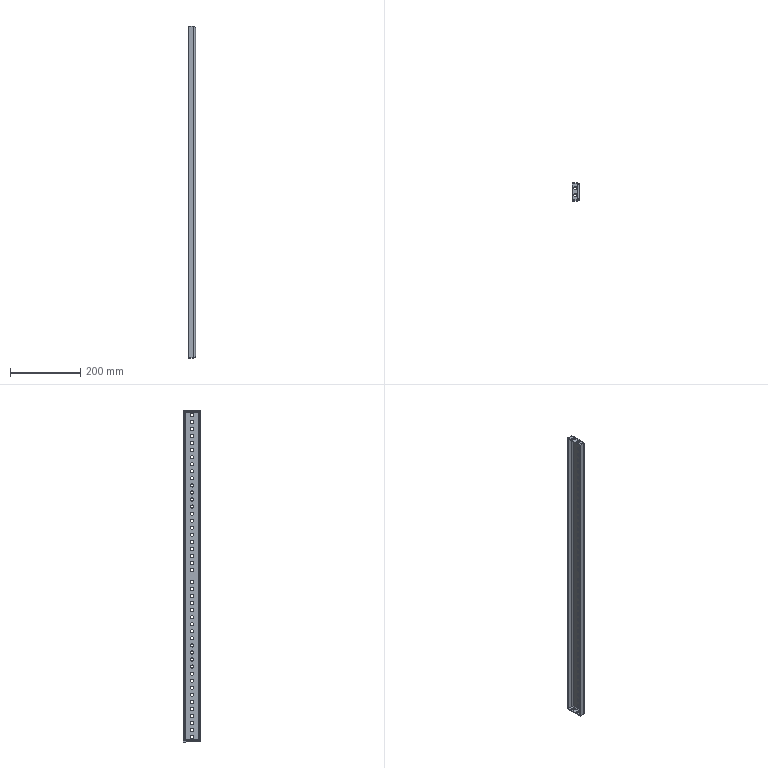Component | SolidWorks | SupportBeamF7-2 | 1 solid | 138 faces | volume 220717 mm3 | cylinder 108 | plane 22 | spline 8 | commonest cylinder face diameters 9 x100 6 x4 12 x4